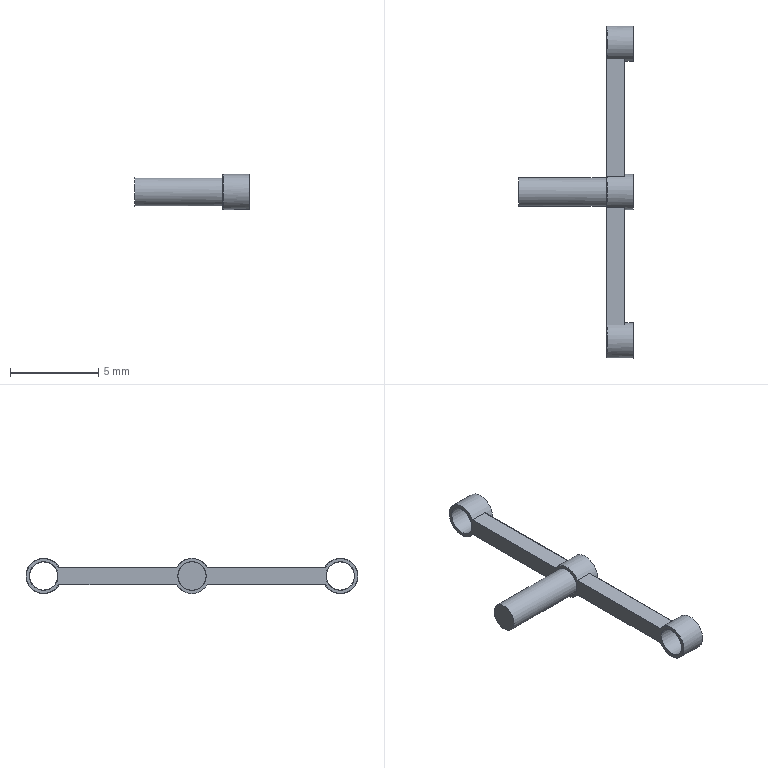Component | NX | CONNECTING_SHAFT_PART_2 | 1 solid | 38 faces | volume 31 mm3 | plane 11 | cylinder 11 | torus 10 | spline 6 | commonest cylinder face diameters 0.02 x5 2 x3 1.6 x3